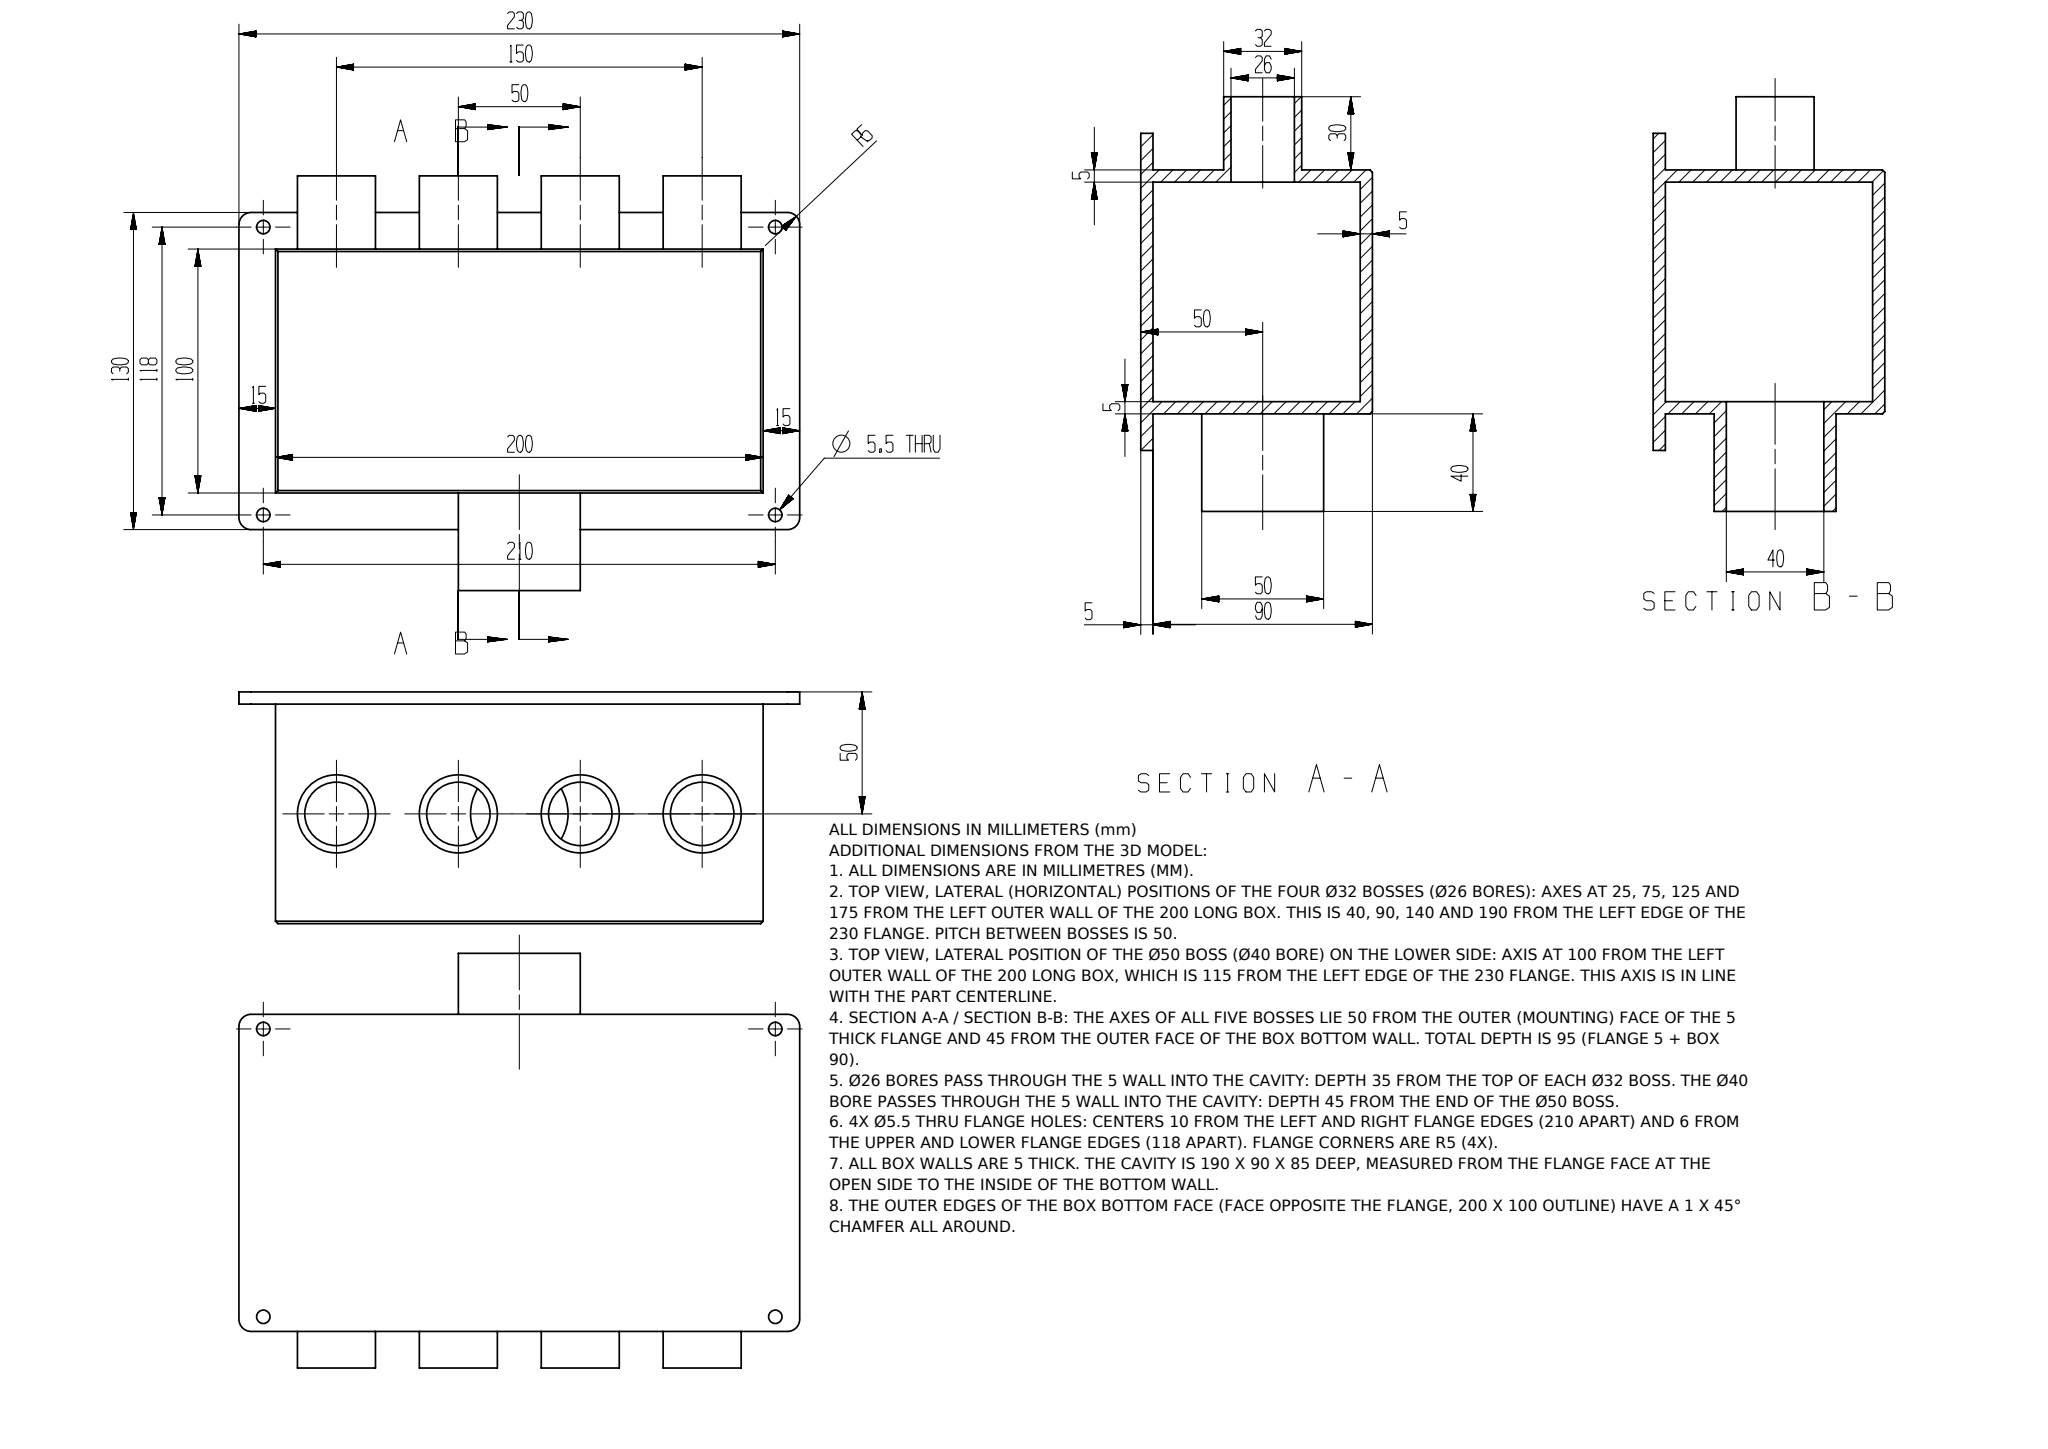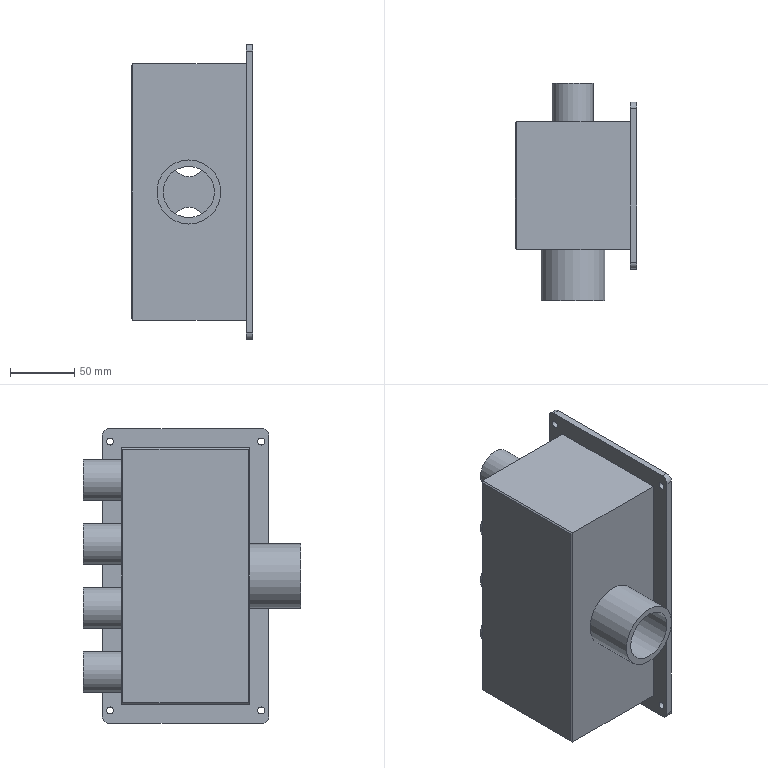Part | NX | mm | 1 solid | 44 faces | box 95 x 170 x 230 mm | volume 539290 mm3 | plane 26 | cylinder 18 | commonest cylinder face diameters 32 x4 26 x4 5.5 x4 10 x4 50 x1 40 x1